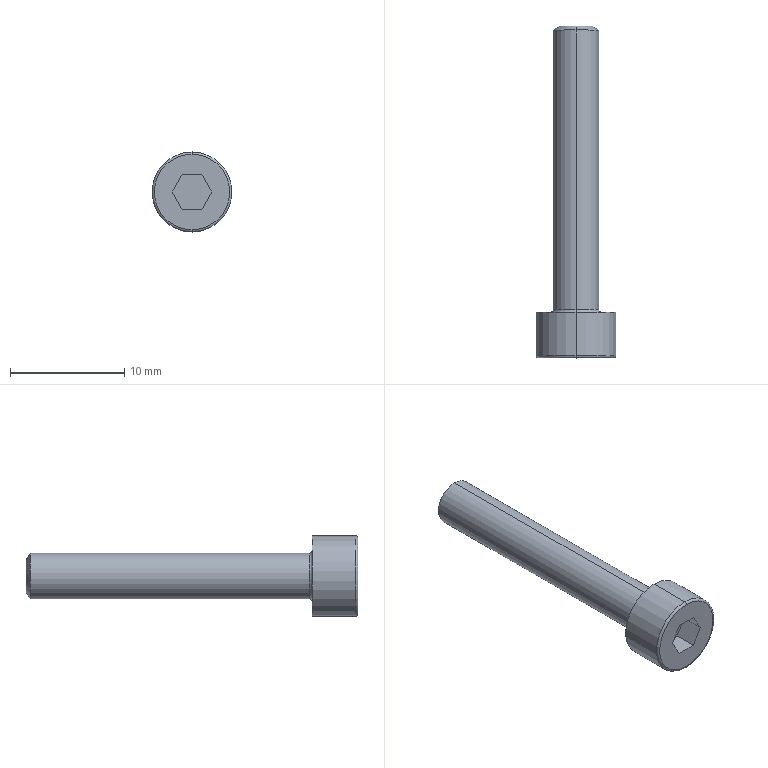Component | NX | HEX_SOCKET_SCREW_M4X25 | 1 solid | 20 faces | volume 451 mm3 | plane 10 | torus 4 | cylinder 4 | cone 2 | commonest cylinder face diameters 7 x2 4 x2